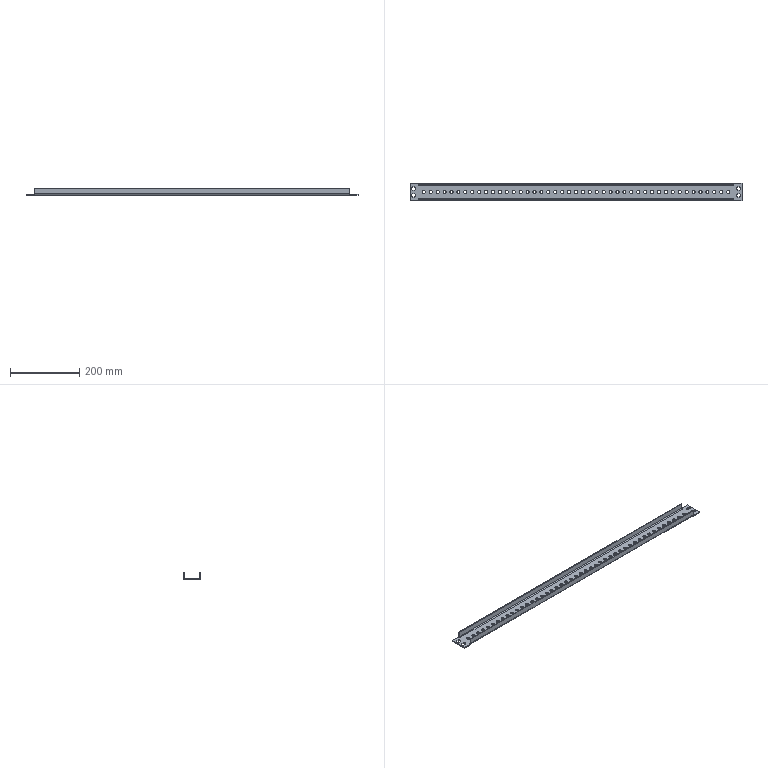Component | SolidWorks | BeamF1-18 | 1 solid | 140 faces | volume 217554 mm3 | cylinder 106 | plane 34 | commonest cylinder face diameters 9 x102 11 x2 5 x2